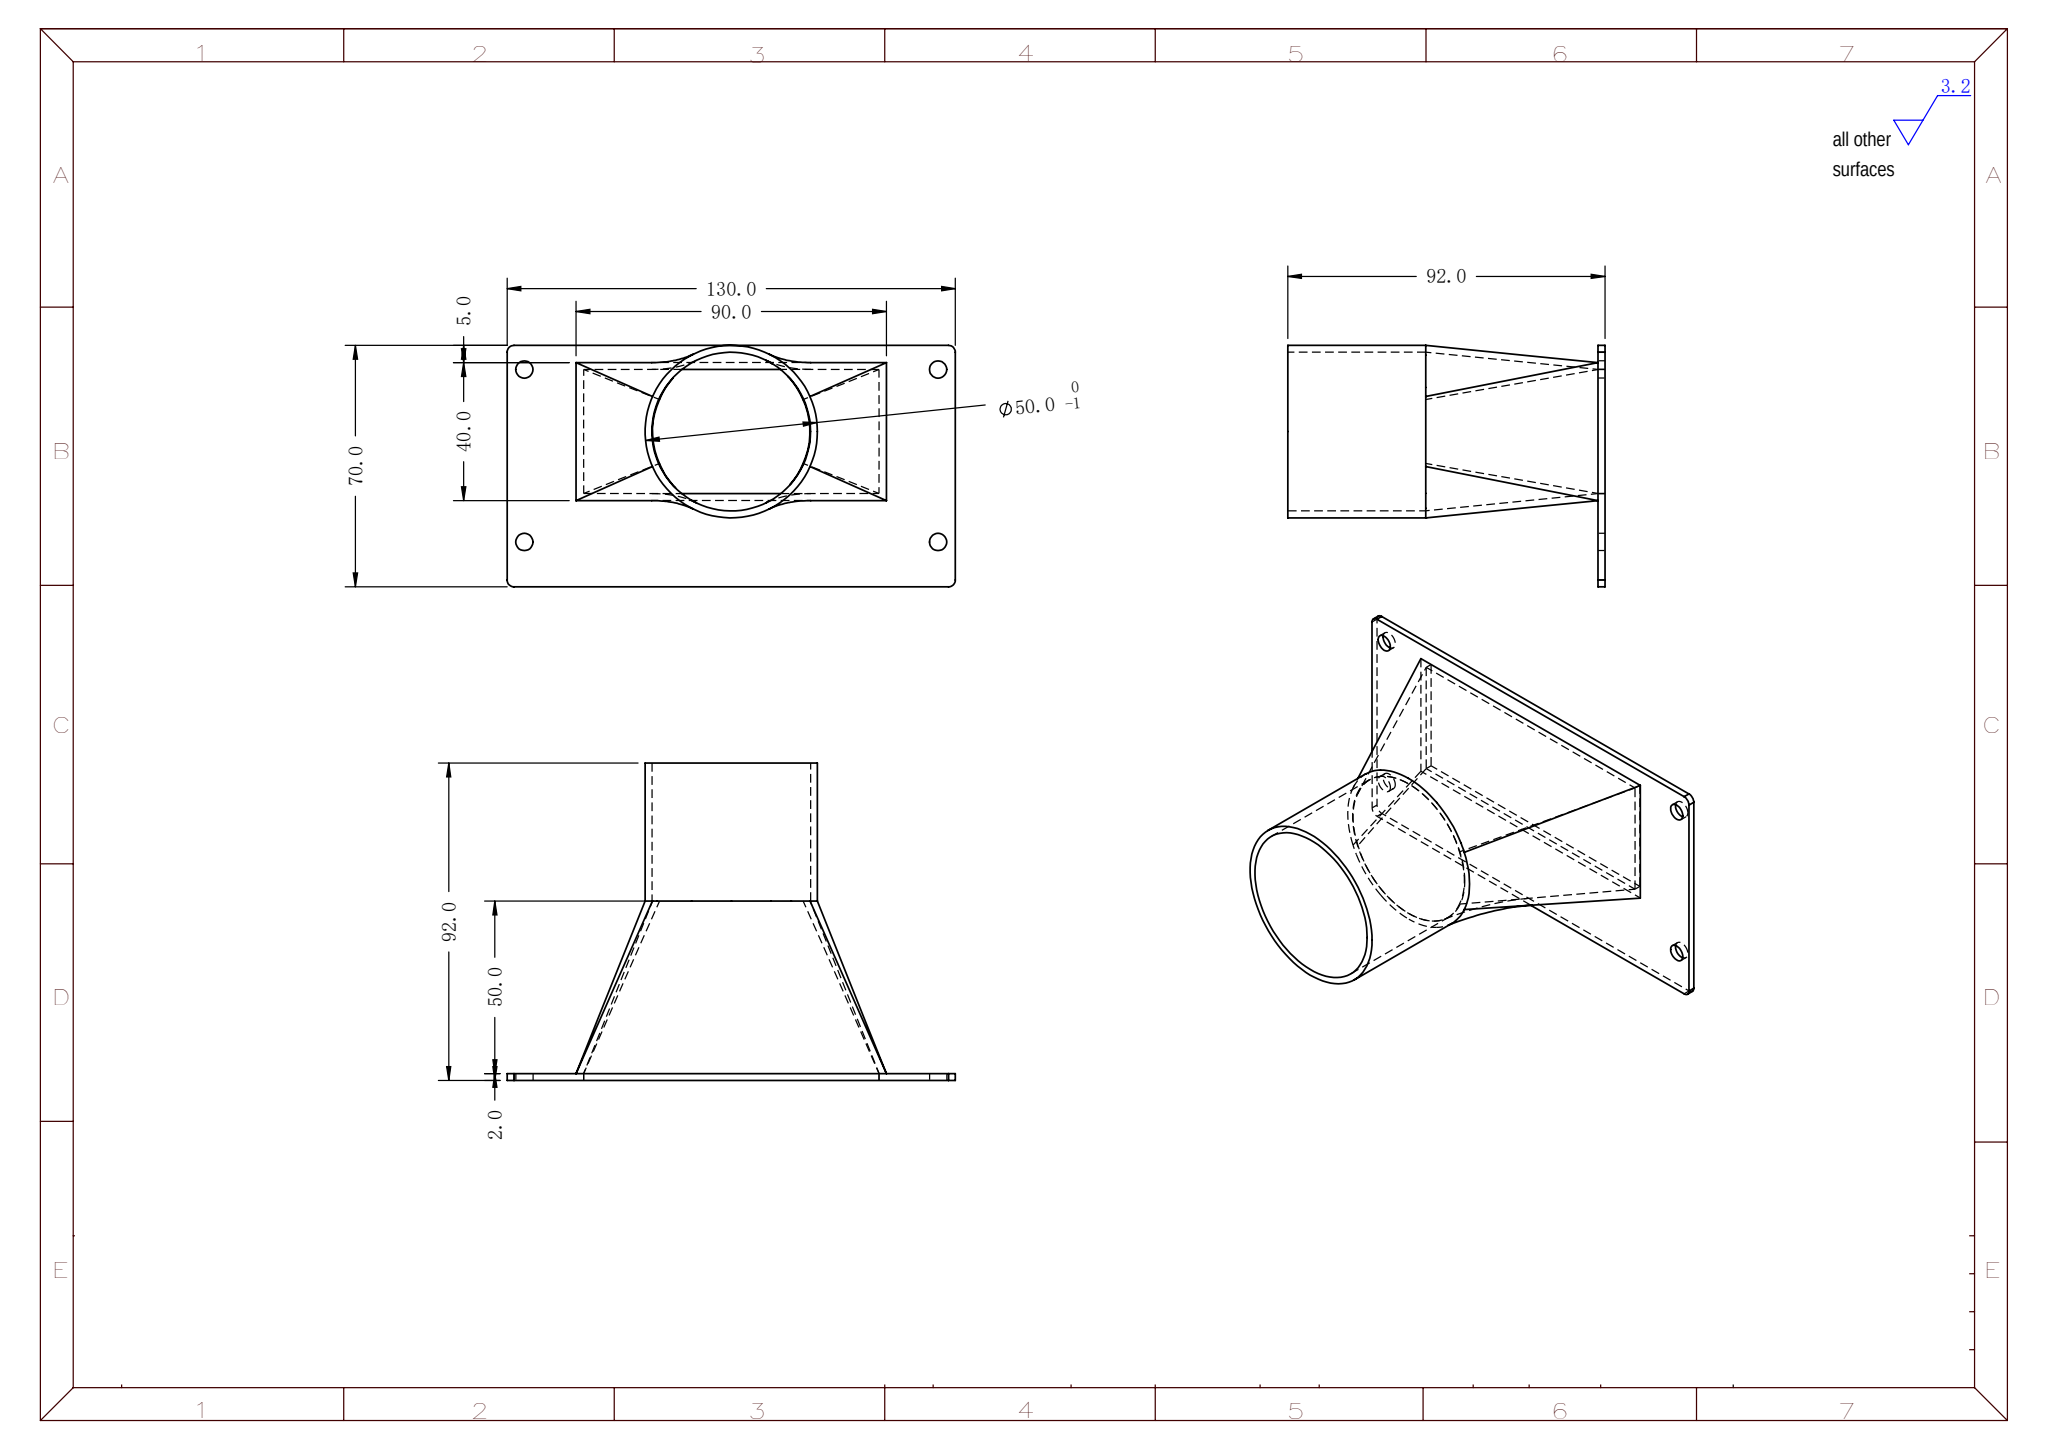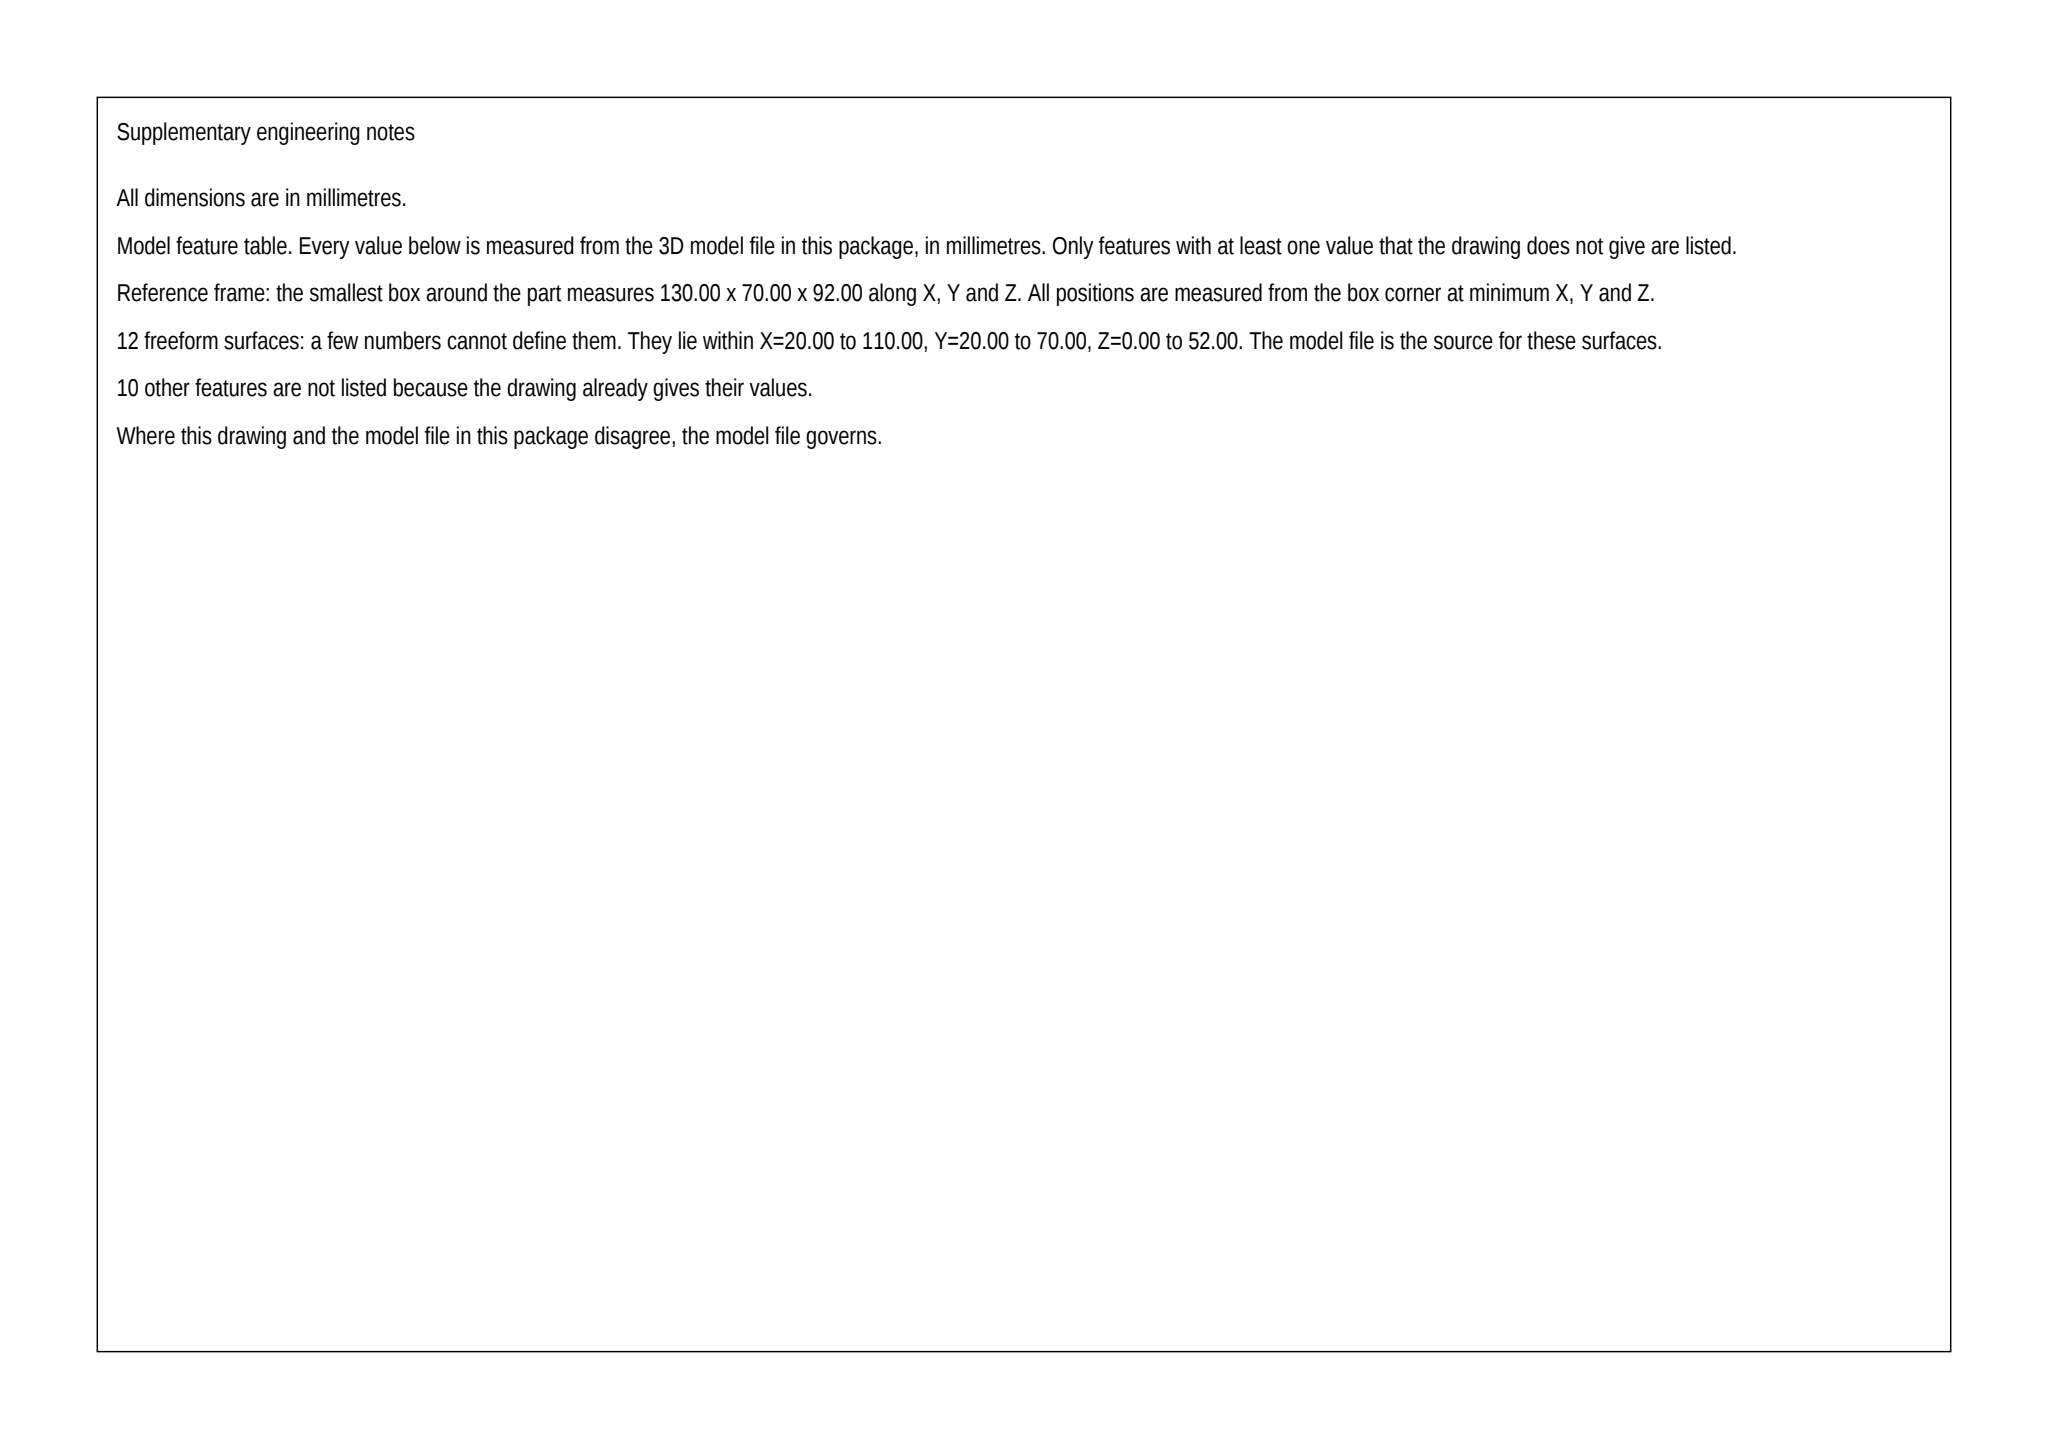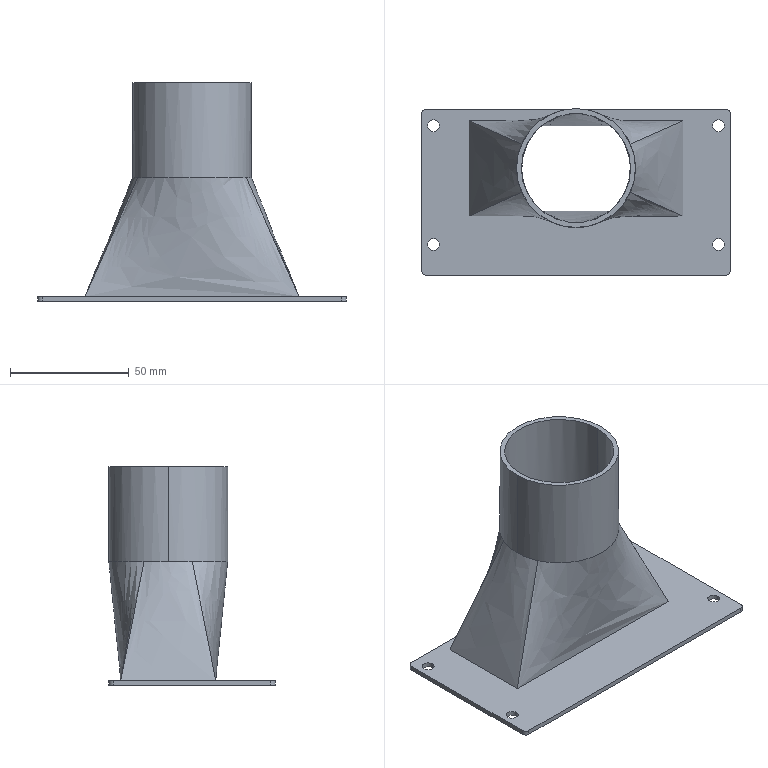Part | SolidWorks | mm | material SUS304 | 1 solid | 36 faces | box 130 x 70 x 92 mm | volume 44131 mm3 | cylinder 16 | spline 12 | plane 8 | commonest cylinder face diameters 5 x8 4 x4 46 x2 50 x2